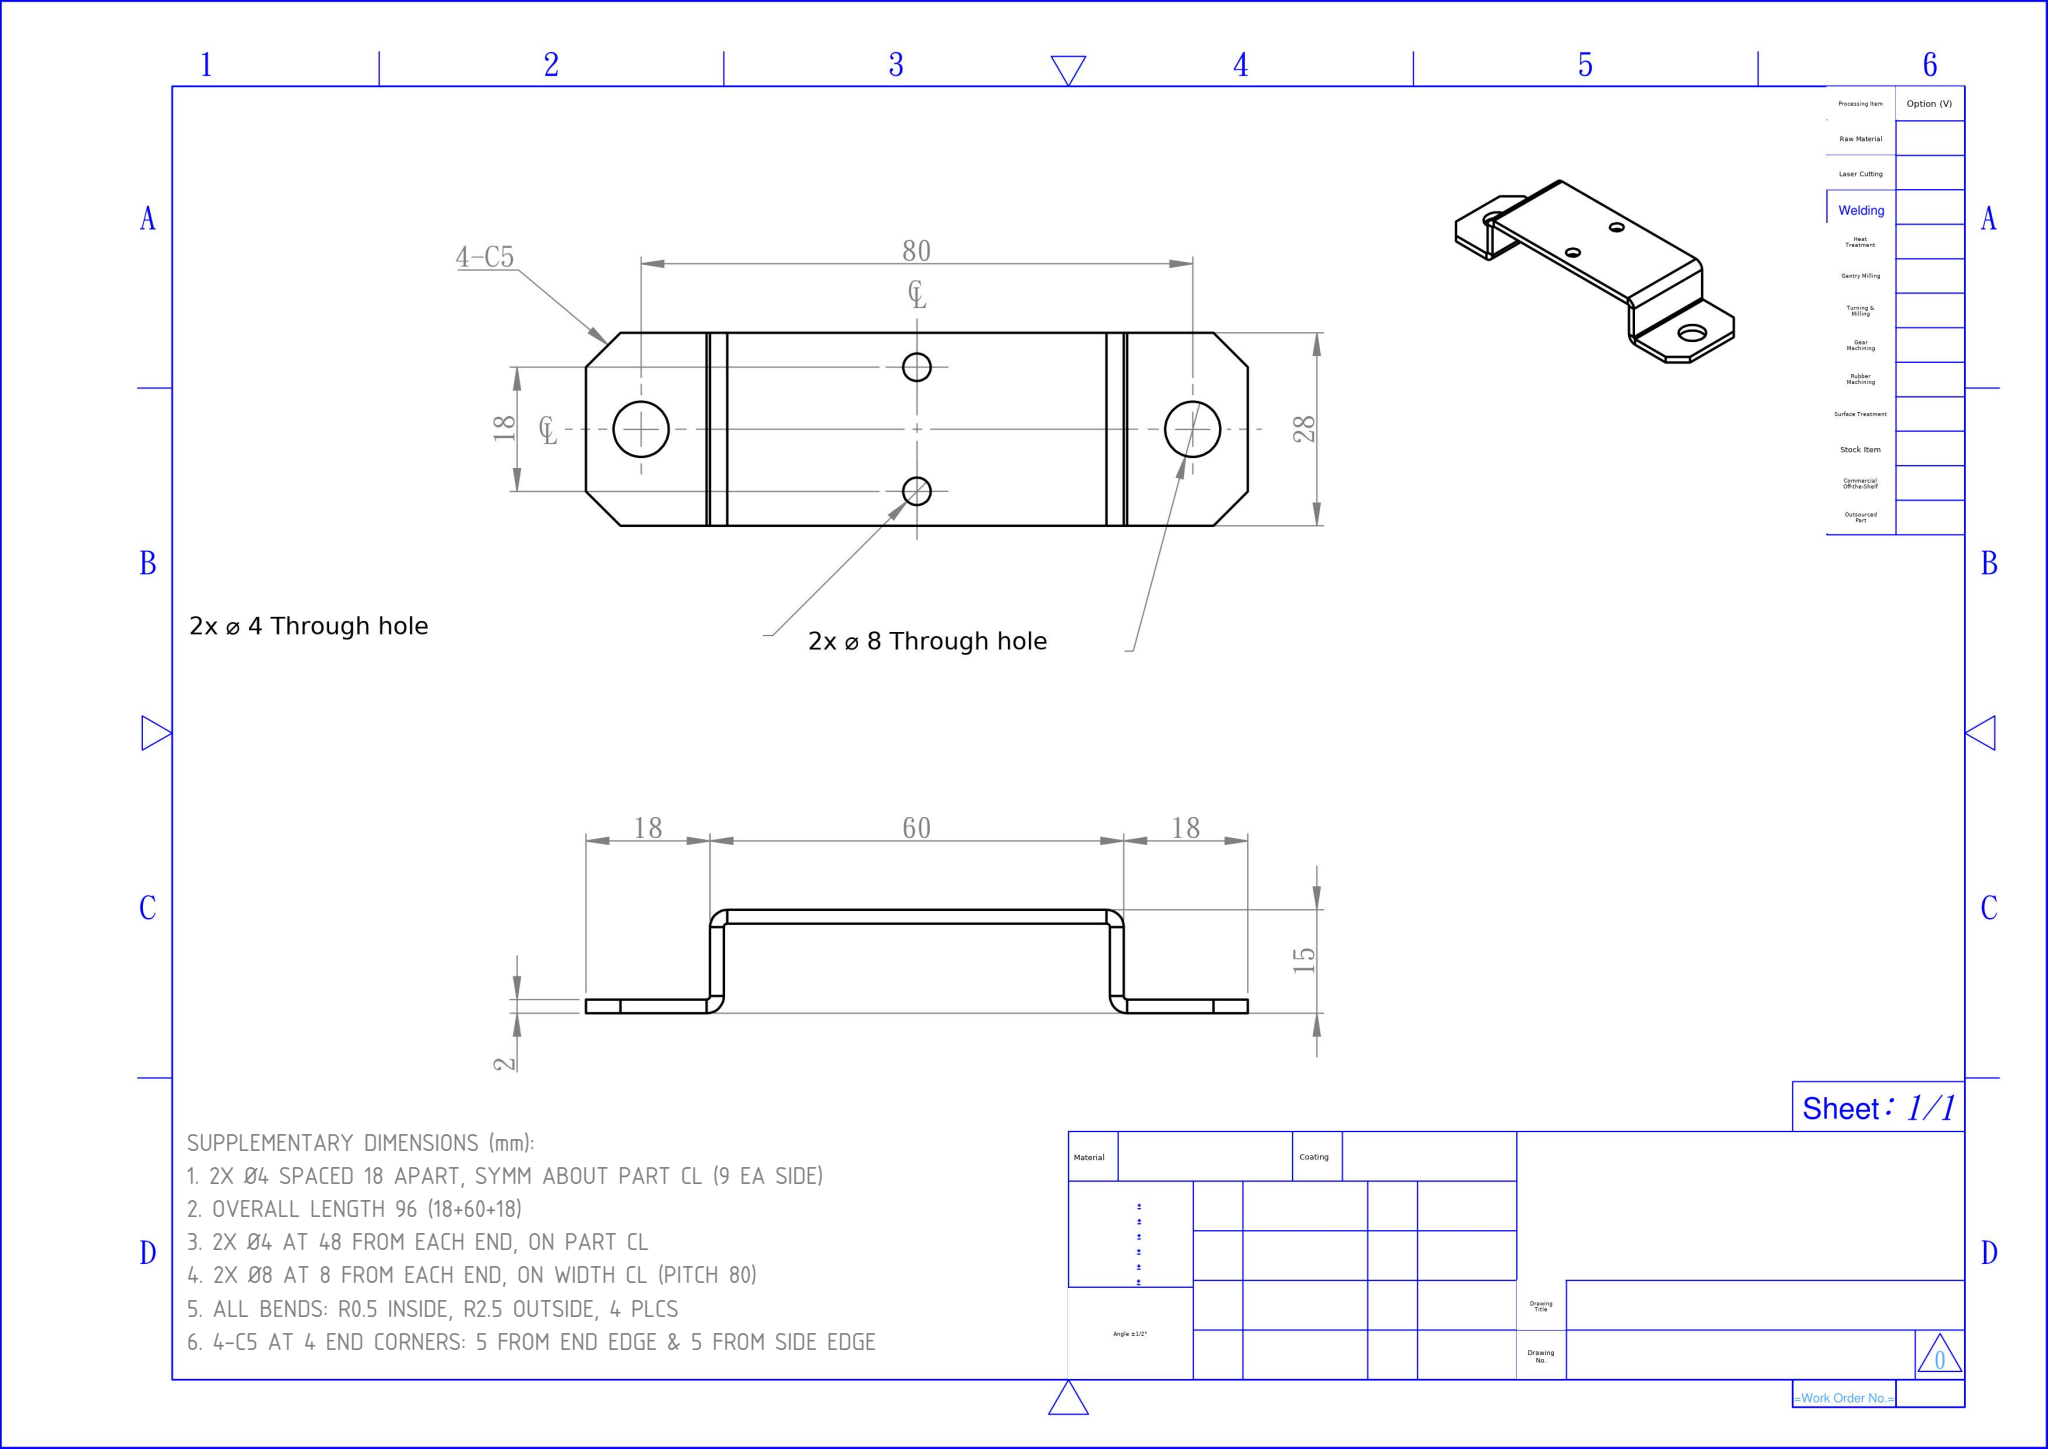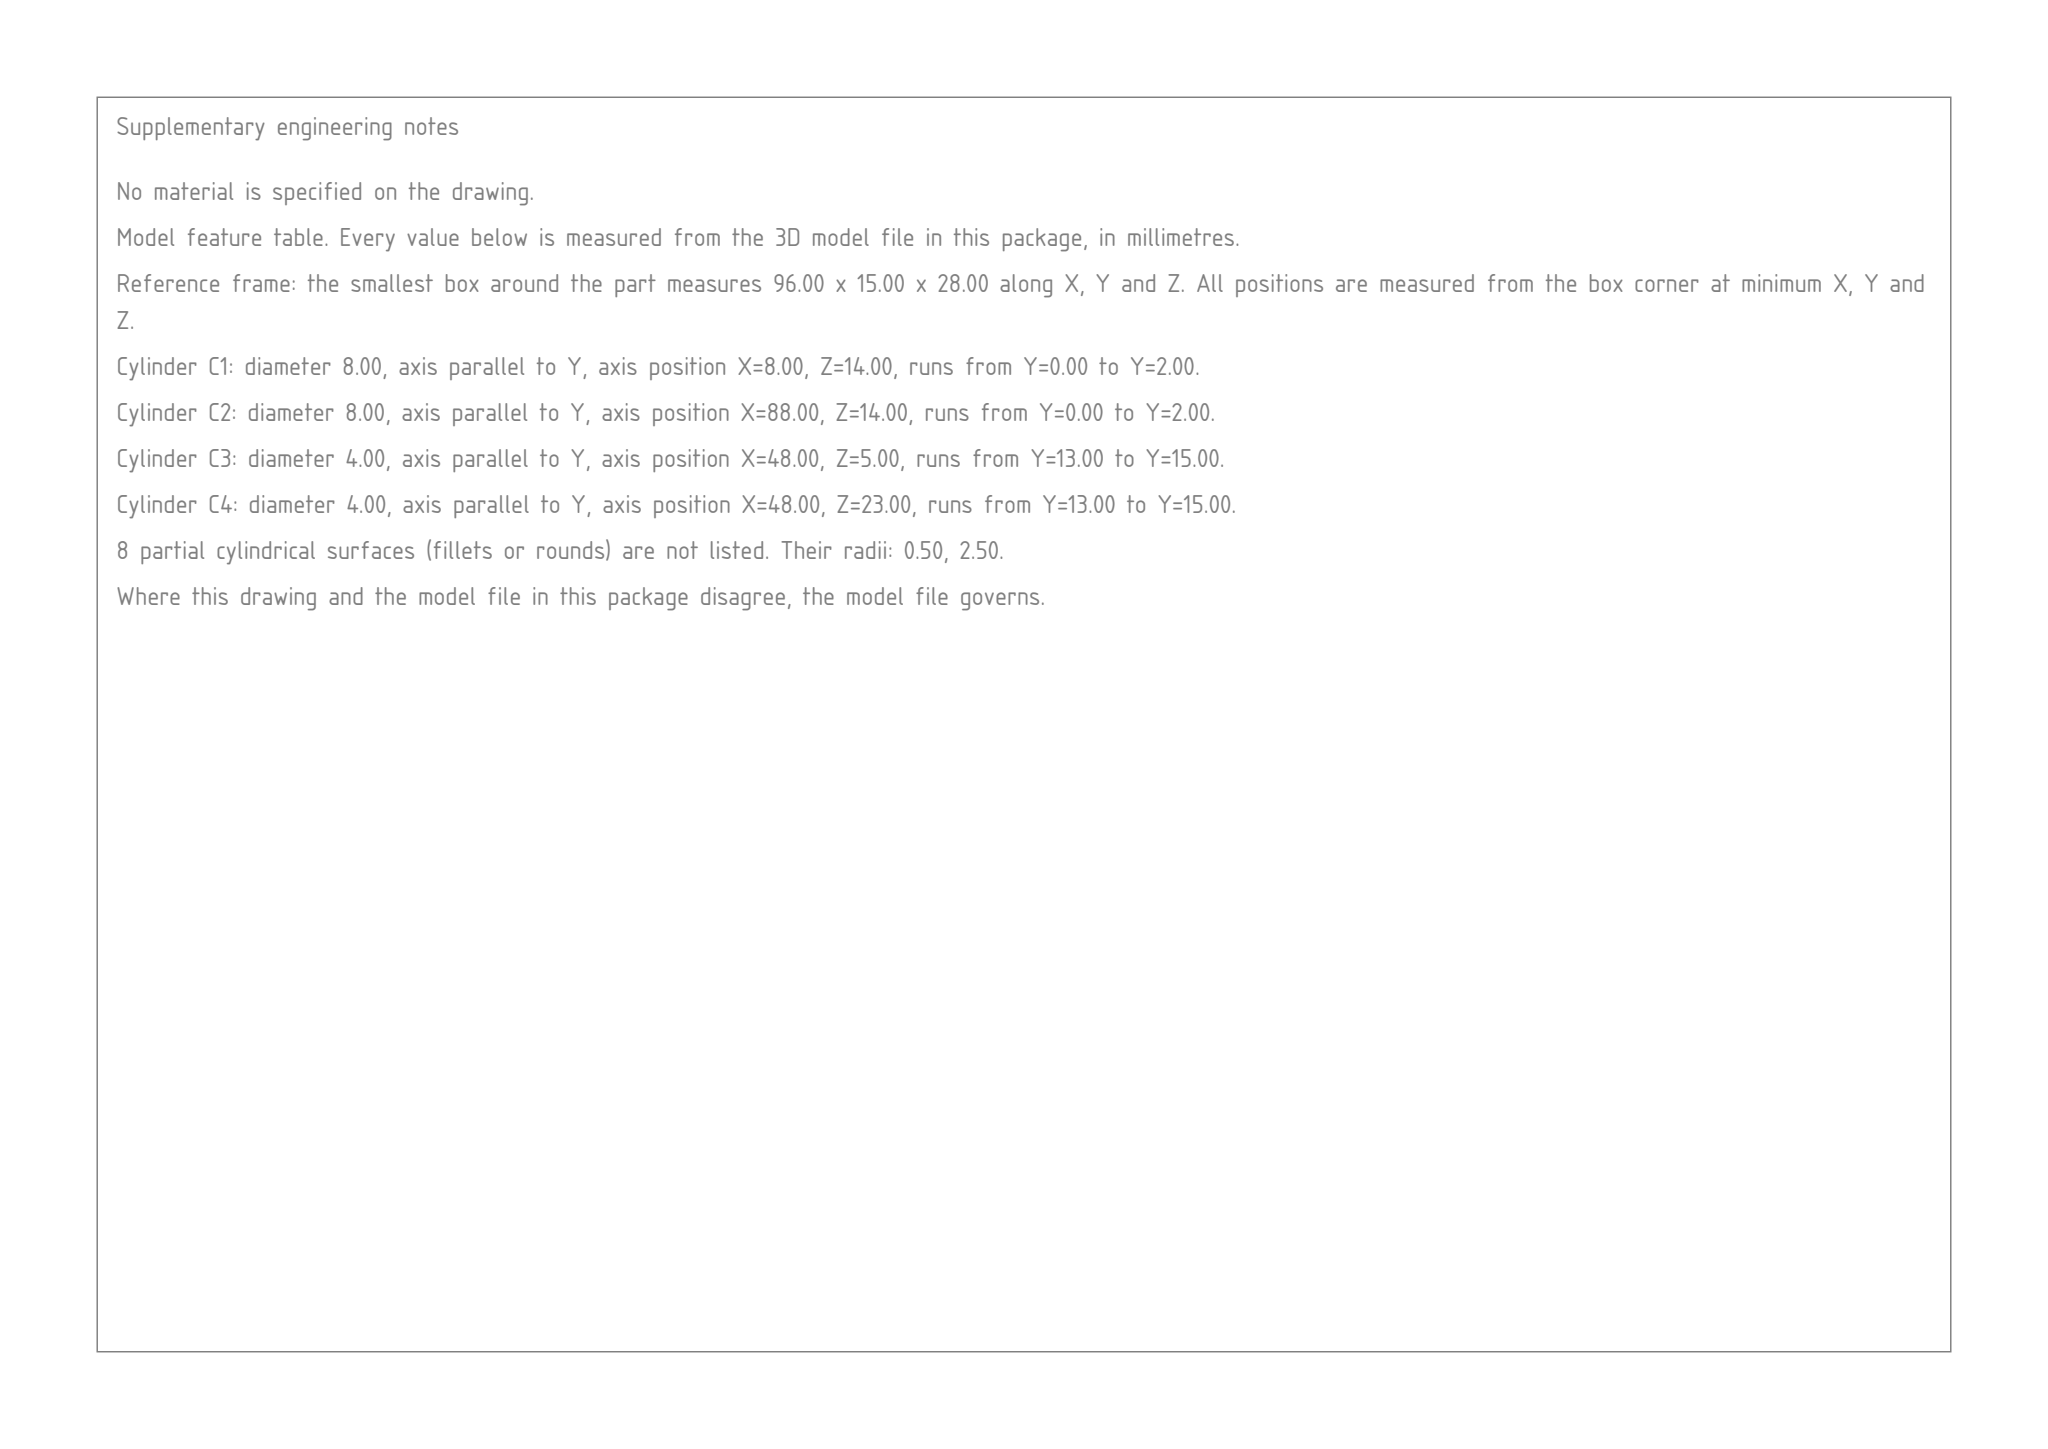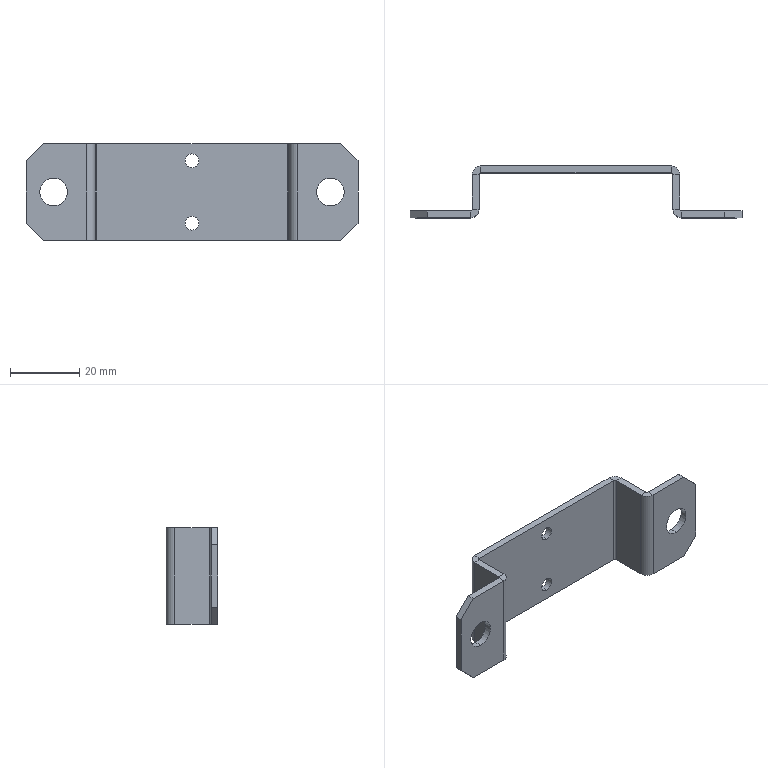Part | SolidWorks | mm | 1 solid | 50 faces | box 96 x 15 x 28 mm | volume 6336 mm3 | plane 34 | cylinder 16 | commonest cylinder face diameters 4 x4 8 x4 5 x4 1 x4